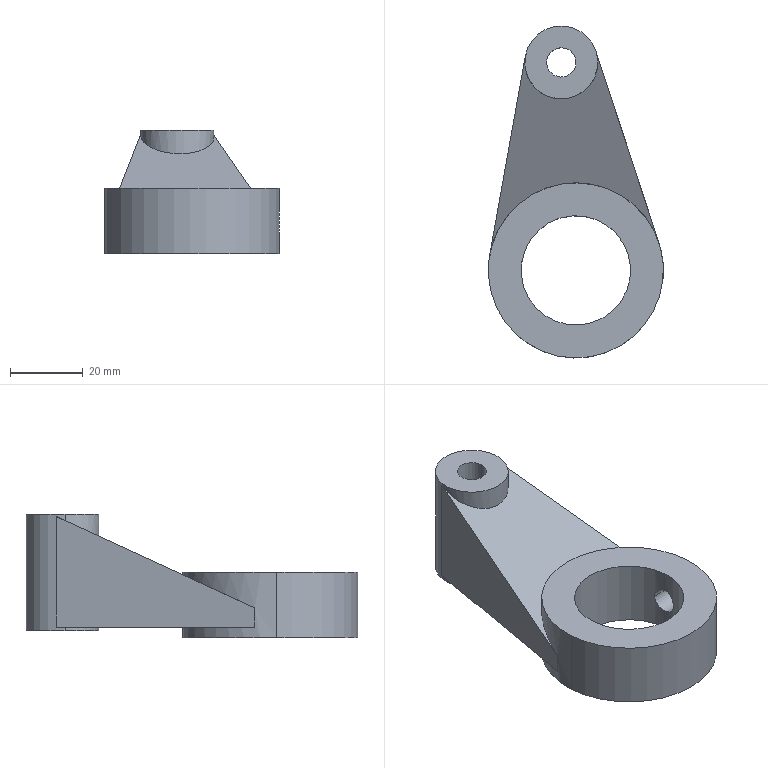Component | SolidWorks | 15Lever-1 | 1 solid | 26 faces | box 48 x 91 x 34 mm | volume 35312 mm3 | cylinder 13 | plane 13 | commonest cylinder face diameters 20 x3 6.8 x2 14.5 x2 30 x2 48 x2 8.02 x2
STEP:
#1=COLOUR_RGB('',0.7922,0.8196,0.9333);
#2=FILL_AREA_STYLE_COLOUR('',#1);
#3=FILL_AREA_STYLE('',(#2));
#4=SURFACE_STYLE_FILL_AREA(#3);
#5=SURFACE_SIDE_STYLE('',(#4));
#6=SURFACE_STYLE_USAGE(.BOTH.,#5);
#7=PRESENTATION_STYLE_ASSIGNMENT((#6));
#8=CARTESIAN_POINT('',(2.078,-2.267,14.724));
#9=VERTEX_POINT('',#8);
#10=CARTESIAN_POINT('',(2.083,-2.133,14.591));
#11=VERTEX_POINT('',#10);
#12=CARTESIAN_POINT('',(2.078,-2.267,14.724));
#13=CARTESIAN_POINT('',(2.078,-2.267,14.716));
#14=CARTESIAN_POINT('',(2.078,-2.267,14.707));
#15=CARTESIAN_POINT('',(2.078,-2.263,14.69));
#16=CARTESIAN_POINT('',(2.079,-2.26,14.681));
#17=CARTESIAN_POINT('',(2.08,-2.254,14.665));
#18=CARTESIAN_POINT('',(2.08,-2.25,14.657));
#19=CARTESIAN_POINT('',(2.081,-2.24,14.643));
#20=CARTESIAN_POINT('',(2.082,-2.234,14.636));
#21=CARTESIAN_POINT('',(2.083,-2.222,14.624));
#22=CARTESIAN_POINT('',(2.084,-2.215,14.618));
#23=CARTESIAN_POINT('',(2.084,-2.2,14.608));
#24=CARTESIAN_POINT('',(2.085,-2.192,14.604));
#25=CARTESIAN_POINT('',(2.085,-2.176,14.597));
#26=CARTESIAN_POINT('',(2.085,-2.168,14.595));
#27=CARTESIAN_POINT('',(2.085,-2.15,14.591));
#28=CARTESIAN_POINT('',(2.084,-2.142,14.591));
#29=CARTESIAN_POINT('',(2.083,-2.133,14.591));
#30=B_SPLINE_CURVE_WITH_KNOTS('',3,(#12,#13,#14,#15,#16,#17,#18,#19,#20,#21,#22,#23,#24,#25,#26,#27,#28,#29),.UNSPECIFIED.,.F.,.F.,(4,2,2,2,2,2,2,2,4),(0.016,0.01666,0.01733,0.018,0.01866,0.01933,0.01999,0.02066,0.02133),.UNSPECIFIED.);
#31=EDGE_CURVE('',#9,#11,#30,.T.);
#32=ORIENTED_EDGE('',*,*,#31,.F.);
#33=CARTESIAN_POINT('',(2.437,-2.242,14.724));
#34=VERTEX_POINT('',#33);
#35=CARTESIAN_POINT('',(2.446,-2.242,14.724));
#36=DIRECTION('',(0.9975,0.07,0.));
#37=VECTOR('',#36,39.37);
#38=LINE('',#35,#37);
#39=EDGE_CURVE('',#9,#34,#38,.T.);
#40=ORIENTED_EDGE('',*,*,#39,.T.);
#41=CARTESIAN_POINT('',(2.437,-2.108,14.591));
#42=VERTEX_POINT('',#41);
#43=CARTESIAN_POINT('',(2.437,-2.242,14.724));
#44=CARTESIAN_POINT('',(2.437,-2.242,14.716));
#45=CARTESIAN_POINT('',(2.437,-2.241,14.707));
#46=CARTESIAN_POINT('',(2.437,-2.238,14.69));
#47=CARTESIAN_POINT('',(2.437,-2.235,14.681));
#48=CARTESIAN_POINT('',(2.438,-2.229,14.665));
#49=CARTESIAN_POINT('',(2.438,-2.224,14.657));
#50=CARTESIAN_POINT('',(2.438,-2.215,14.643));
#51=CARTESIAN_POINT('',(2.439,-2.209,14.636));
#52=CARTESIAN_POINT('',(2.439,-2.197,14.624));
#53=CARTESIAN_POINT('',(2.439,-2.19,14.618));
#54=CARTESIAN_POINT('',(2.439,-2.175,14.608));
#55=CARTESIAN_POINT('',(2.439,-2.167,14.604));
#56=CARTESIAN_POINT('',(2.439,-2.151,14.597));
#57=CARTESIAN_POINT('',(2.439,-2.143,14.595));
#58=CARTESIAN_POINT('',(2.438,-2.126,14.591));
#59=CARTESIAN_POINT('',(2.438,-2.117,14.591));
#60=CARTESIAN_POINT('',(2.437,-2.108,14.591));
#61=B_SPLINE_CURVE_WITH_KNOTS('',3,(#43,#44,#45,#46,#47,#48,#49,#50,#51,#52,#53,#54,#55,#56,#57,#58,#59,#60),.UNSPECIFIED.,.F.,.F.,(4,2,2,2,2,2,2,2,4),(0.01064,0.01131,0.01197,0.01264,0.0133,0.01397,0.01464,0.0153,0.01597),.UNSPECIFIED.);
#62=EDGE_CURVE('',#34,#42,#61,.T.);
#63=ORIENTED_EDGE('',*,*,#62,.T.);
#64=CARTESIAN_POINT('',(2.418,-1.975,14.724));
#65=VERTEX_POINT('',#64);
#66=CARTESIAN_POINT('',(2.437,-2.108,14.591));
#67=CARTESIAN_POINT('',(2.436,-2.099,14.591));
#68=CARTESIAN_POINT('',(2.436,-2.091,14.591));
#69=CARTESIAN_POINT('',(2.434,-2.073,14.595));
#70=CARTESIAN_POINT('',(2.433,-2.065,14.597));
#71=CARTESIAN_POINT('',(2.431,-2.049,14.604));
#72=CARTESIAN_POINT('',(2.43,-2.041,14.608));
#73=CARTESIAN_POINT('',(2.428,-2.027,14.618));
#74=CARTESIAN_POINT('',(2.427,-2.02,14.624));
#75=CARTESIAN_POINT('',(2.425,-2.008,14.636));
#76=CARTESIAN_POINT('',(2.424,-2.002,14.643));
#77=CARTESIAN_POINT('',(2.422,-1.993,14.657));
#78=CARTESIAN_POINT('',(2.421,-1.989,14.665));
#79=CARTESIAN_POINT('',(2.42,-1.982,14.681));
#80=CARTESIAN_POINT('',(2.419,-1.979,14.69));
#81=CARTESIAN_POINT('',(2.418,-1.976,14.707));
#82=CARTESIAN_POINT('',(2.418,-1.975,14.716));
#83=CARTESIAN_POINT('',(2.418,-1.975,14.724));
#84=B_SPLINE_CURVE_WITH_KNOTS('',3,(#66,#67,#68,#69,#70,#71,#72,#73,#74,#75,#76,#77,#78,#79,#80,#81,#82,#83),.UNSPECIFIED.,.F.,.F.,(4,2,2,2,2,2,2,2,4),(0.01597,0.01663,0.0173,0.01796,0.01863,0.01929,0.01995,0.02062,0.02128),.UNSPECIFIED.);
#85=EDGE_CURVE('',#42,#65,#84,.T.);
#86=ORIENTED_EDGE('',*,*,#85,.T.);
#87=CARTESIAN_POINT('',(2.059,-2.,14.724));
#88=VERTEX_POINT('',#87);
#89=CARTESIAN_POINT('',(2.428,-1.974,14.724));
#90=DIRECTION('',(0.9975,0.07,0.));
#91=VECTOR('',#90,39.37);
#92=LINE('',#89,#91);
#93=EDGE_CURVE('',#88,#65,#92,.T.);
#94=ORIENTED_EDGE('',*,*,#93,.F.);
#95=CARTESIAN_POINT('',(2.083,-2.133,14.591));
#96=CARTESIAN_POINT('',(2.083,-2.124,14.591));
#97=CARTESIAN_POINT('',(2.082,-2.115,14.591));
#98=CARTESIAN_POINT('',(2.08,-2.098,14.595));
#99=CARTESIAN_POINT('',(2.079,-2.09,14.597));
#100=CARTESIAN_POINT('',(2.076,-2.074,14.604));
#101=CARTESIAN_POINT('',(2.075,-2.066,14.608));
#102=CARTESIAN_POINT('',(2.072,-2.052,14.618));
#103=CARTESIAN_POINT('',(2.071,-2.045,14.624));
#104=CARTESIAN_POINT('',(2.068,-2.033,14.636));
#105=CARTESIAN_POINT('',(2.066,-2.027,14.643));
#106=CARTESIAN_POINT('',(2.064,-2.018,14.657));
#107=CARTESIAN_POINT('',(2.063,-2.014,14.665));
#108=CARTESIAN_POINT('',(2.061,-2.007,14.681));
#109=CARTESIAN_POINT('',(2.06,-2.005,14.69));
#110=CARTESIAN_POINT('',(2.059,-2.001,14.707));
#111=CARTESIAN_POINT('',(2.059,-2.,14.716));
#112=CARTESIAN_POINT('',(2.059,-2.,14.724));
#113=B_SPLINE_CURVE_WITH_KNOTS('',3,(#95,#96,#97,#98,#99,#100,#101,#102,#103,#104,#105,#106,#107,#108,#109,#110,#111,#112),.UNSPECIFIED.,.F.,.F.,(4,2,2,2,2,2,2,2,4),(0.,0.0006667,0.001333,0.002,0.002667,0.003334,0.004,0.004667,0.005334),.UNSPECIFIED.);
#114=EDGE_CURVE('',#11,#88,#113,.T.);
#115=ORIENTED_EDGE('',*,*,#114,.F.);
#116=EDGE_LOOP('',(#32,#40,#63,#86,#94,#115));
#117=FACE_OUTER_BOUND('',#116,.T.);
#118=CARTESIAN_POINT('',(2.437,-2.108,14.724));
#119=DIRECTION('',(0.9975,0.07,0.));
#120=DIRECTION('',(-0.07,0.9975,0.));
#121=AXIS2_PLACEMENT_3D('',#118,#119,#120);
#122=CYLINDRICAL_SURFACE('',#121,0.1339);
#123=ADVANCED_FACE('',(#117),#122,.F.);
#124=CARTESIAN_POINT('',(1.622,0.0899,15.433));
#125=VERTEX_POINT('',#124);
#126=CARTESIAN_POINT('',(1.052,0.04993,15.433));
#127=VERTEX_POINT('',#126);
#128=CARTESIAN_POINT('',(1.337,0.06992,15.433));
#129=DIRECTION('',(0.,-0.,-1.));
#130=DIRECTION('',(-0.9975,-0.07,0.));
#131=AXIS2_PLACEMENT_3D('',#128,#129,#130);
#132=CIRCLE('',#131,0.2854);
#133=EDGE_CURVE('',#125,#127,#132,.T.);
#134=ORIENTED_EDGE('',*,*,#133,.F.);
#135=CARTESIAN_POINT('',(1.622,0.0899,14.449));
#136=VERTEX_POINT('',#135);
#137=CARTESIAN_POINT('',(1.622,0.0899,15.433));
#138=DIRECTION('',(0.,-0.,-1.));
#139=VECTOR('',#138,39.37);
#140=LINE('',#137,#139);
#141=EDGE_CURVE('',#125,#136,#140,.T.);
#142=ORIENTED_EDGE('',*,*,#141,.T.);
#143=CARTESIAN_POINT('',(1.052,0.04993,14.449));
#144=VERTEX_POINT('',#143);
#145=CARTESIAN_POINT('',(1.337,0.06992,14.449));
#146=DIRECTION('',(0.,-0.,-1.));
#147=DIRECTION('',(-0.9975,-0.07,0.));
#148=AXIS2_PLACEMENT_3D('',#145,#146,#147);
#149=CIRCLE('',#148,0.2854);
#150=EDGE_CURVE('',#136,#144,#149,.T.);
#151=ORIENTED_EDGE('',*,*,#150,.T.);
#152=CARTESIAN_POINT('',(1.052,0.04993,15.433));
#153=DIRECTION('',(0.,-0.,-1.));
#154=VECTOR('',#153,39.37);
#155=LINE('',#152,#154);
#156=EDGE_CURVE('',#127,#144,#155,.T.);
#157=ORIENTED_EDGE('',*,*,#156,.F.);
#158=EDGE_LOOP('',(#134,#142,#151,#157));
#159=FACE_OUTER_BOUND('',#158,.T.);
#160=CARTESIAN_POINT('',(1.337,0.06992,15.433));
#161=DIRECTION('',(0.,-0.,-1.));
#162=DIRECTION('',(-0.9975,-0.07,0.));
#163=AXIS2_PLACEMENT_3D('',#160,#161,#162);
#164=CYLINDRICAL_SURFACE('',#163,0.2854);
#165=ADVANCED_FACE('',(#159),#164,.F.);
#166=CARTESIAN_POINT('',(0.9053,-2.216,14.37));
#167=VERTEX_POINT('',#166);
#168=CARTESIAN_POINT('',(2.083,-2.133,14.37));
#169=VERTEX_POINT('',#168);
#170=CARTESIAN_POINT('',(1.494,-2.174,14.37));
#171=DIRECTION('',(-0.,0.,1.));
#172=DIRECTION('',(0.9975,0.07,0.));
#173=AXIS2_PLACEMENT_3D('',#170,#171,#172);
#174=CIRCLE('',#173,0.5906);
#175=EDGE_CURVE('',#167,#169,#174,.T.);
#176=ORIENTED_EDGE('',*,*,#175,.F.);
#177=CARTESIAN_POINT('',(0.9053,-2.216,15.079));
#178=VERTEX_POINT('',#177);
#179=CARTESIAN_POINT('',(0.9053,-2.216,14.37));
#180=DIRECTION('',(-0.,0.,1.));
#181=VECTOR('',#180,39.37);
#182=LINE('',#179,#181);
#183=EDGE_CURVE('',#167,#178,#182,.T.);
#184=ORIENTED_EDGE('',*,*,#183,.T.);
#185=CARTESIAN_POINT('',(2.083,-2.133,15.079));
#186=VERTEX_POINT('',#185);
#187=CARTESIAN_POINT('',(1.494,-2.174,15.079));
#188=DIRECTION('',(0.,-0.,-1.));
#189=DIRECTION('',(-0.9975,-0.07,0.));
#190=AXIS2_PLACEMENT_3D('',#187,#188,#189);
#191=CIRCLE('',#190,0.5906);
#192=EDGE_CURVE('',#186,#178,#191,.T.);
#193=ORIENTED_EDGE('',*,*,#192,.F.);
#194=CARTESIAN_POINT('',(2.083,-2.133,14.858));
#195=VERTEX_POINT('',#194);
#196=CARTESIAN_POINT('',(2.083,-2.133,14.37));
#197=DIRECTION('',(-0.,0.,1.));
#198=VECTOR('',#197,39.37);
#199=LINE('',#196,#198);
#200=EDGE_CURVE('',#195,#186,#199,.T.);
#201=ORIENTED_EDGE('',*,*,#200,.F.);
#202=CARTESIAN_POINT('',(2.083,-2.133,14.858));
#203=CARTESIAN_POINT('',(2.084,-2.142,14.858));
#204=CARTESIAN_POINT('',(2.085,-2.15,14.857));
#205=CARTESIAN_POINT('',(2.085,-2.168,14.854));
#206=CARTESIAN_POINT('',(2.085,-2.176,14.851));
#207=CARTESIAN_POINT('',(2.085,-2.192,14.845));
#208=CARTESIAN_POINT('',(2.084,-2.2,14.841));
#209=CARTESIAN_POINT('',(2.084,-2.215,14.831));
#210=CARTESIAN_POINT('',(2.083,-2.222,14.825));
#211=CARTESIAN_POINT('',(2.082,-2.234,14.813));
#212=CARTESIAN_POINT('',(2.081,-2.24,14.806));
#213=CARTESIAN_POINT('',(2.08,-2.249,14.792));
#214=CARTESIAN_POINT('',(2.08,-2.254,14.784));
#215=CARTESIAN_POINT('',(2.078,-2.264,14.76));
#216=CARTESIAN_POINT('',(2.078,-2.267,14.742));
#217=CARTESIAN_POINT('',(2.078,-2.267,14.724));
#218=B_SPLINE_CURVE_WITH_KNOTS('',3,(#202,#203,#204,#205,#206,#207,#208,#209,#210,#211,#212,#213,#214,#215,#216,#217),.UNSPECIFIED.,.F.,.F.,(4,2,2,2,2,2,2,4),(0.01066,0.01133,0.012,0.01266,0.01333,0.014,0.01466,0.016),.UNSPECIFIED.);
#219=EDGE_CURVE('',#195,#9,#218,.T.);
#220=ORIENTED_EDGE('',*,*,#219,.T.);
#221=ORIENTED_EDGE('',*,*,#31,.T.);
#222=CARTESIAN_POINT('',(2.083,-2.133,14.37));
#223=DIRECTION('',(-0.,0.,1.));
#224=VECTOR('',#223,39.37);
#225=LINE('',#222,#224);
#226=EDGE_CURVE('',#169,#11,#225,.T.);
#227=ORIENTED_EDGE('',*,*,#226,.F.);
#228=EDGE_LOOP('',(#176,#184,#193,#201,#220,#221,#227));
#229=FACE_OUTER_BOUND('',#228,.T.);
#230=CARTESIAN_POINT('',(1.494,-2.174,14.37));
#231=DIRECTION('',(-0.,0.,1.));
#232=DIRECTION('',(0.9975,0.07,0.));
#233=AXIS2_PLACEMENT_3D('',#230,#231,#232);
#234=CYLINDRICAL_SURFACE('',#233,0.5906);
#235=ADVANCED_FACE('',(#229),#234,.F.);
#236=CARTESIAN_POINT('',(0.5643,-2.007,14.488));
#237=VERTEX_POINT('',#236);
#238=CARTESIAN_POINT('',(0.86,-1.474,14.488));
#239=VERTEX_POINT('',#238);
#240=CARTESIAN_POINT('',(1.494,-2.174,14.488));
#241=DIRECTION('',(0.,-0.,-1.));
#242=DIRECTION('',(-0.9975,-0.07,0.));
#243=AXIS2_PLACEMENT_3D('',#240,#241,#242);
#244=CIRCLE('',#243,0.9449);
#245=EDGE_CURVE('',#237,#239,#244,.T.);
#246=ORIENTED_EDGE('',*,*,#245,.T.);
#247=CARTESIAN_POINT('',(0.86,-1.474,14.717));
#248=VERTEX_POINT('',#247);
#249=CARTESIAN_POINT('',(0.86,-1.474,16.978));
#250=DIRECTION('',(0.,-0.,-1.));
#251=VECTOR('',#250,39.37);
#252=LINE('',#249,#251);
#253=EDGE_CURVE('',#248,#239,#252,.T.);
#254=ORIENTED_EDGE('',*,*,#253,.F.);
#255=CARTESIAN_POINT('',(2.025,-1.392,14.717));
#256=VERTEX_POINT('',#255);
#257=CARTESIAN_POINT('',(2.025,-1.392,14.717));
#258=CARTESIAN_POINT('',(1.649,-1.137,14.847));
#259=CARTESIAN_POINT('',(1.196,-1.169,14.847));
#260=CARTESIAN_POINT('',(0.86,-1.474,14.717));
#261=(BOUNDED_CURVE()B_SPLINE_CURVE(3,(#257,#258,#259,#260),.UNSPECIFIED.,.F.,.F.)B_SPLINE_CURVE_WITH_KNOTS((4,4),(2.476,3.808),.UNSPECIFIED.)CURVE()GEOMETRIC_REPRESENTATION_ITEM()RATIONAL_B_SPLINE_CURVE((1.,0.8575,0.8575,1.))REPRESENTATION_ITEM(''));
#262=EDGE_CURVE('',#256,#248,#261,.T.);
#263=ORIENTED_EDGE('',*,*,#262,.F.);
#264=CARTESIAN_POINT('',(2.025,-1.392,14.488));
#265=VERTEX_POINT('',#264);
#266=CARTESIAN_POINT('',(2.025,-1.392,16.978));
#267=DIRECTION('',(0.,-0.,-1.));
#268=VECTOR('',#267,39.37);
#269=LINE('',#266,#268);
#270=EDGE_CURVE('',#256,#265,#269,.T.);
#271=ORIENTED_EDGE('',*,*,#270,.T.);
#272=CARTESIAN_POINT('',(2.392,-1.879,14.488));
#273=VERTEX_POINT('',#272);
#274=CARTESIAN_POINT('',(1.494,-2.174,14.488));
#275=DIRECTION('',(0.,-0.,-1.));
#276=DIRECTION('',(-0.9975,-0.07,0.));
#277=AXIS2_PLACEMENT_3D('',#274,#275,#276);
#278=CIRCLE('',#277,0.9449);
#279=EDGE_CURVE('',#265,#273,#278,.T.);
#280=ORIENTED_EDGE('',*,*,#279,.T.);
#281=CARTESIAN_POINT('',(2.392,-1.879,14.695));
#282=VERTEX_POINT('',#281);
#283=CARTESIAN_POINT('',(2.392,-1.879,18.131));
#284=DIRECTION('',(0.,-0.,-1.));
#285=VECTOR('',#284,39.37);
#286=LINE('',#283,#285);
#287=EDGE_CURVE('',#282,#273,#286,.T.);
#288=ORIENTED_EDGE('',*,*,#287,.F.);
#289=CARTESIAN_POINT('',(0.5643,-2.007,14.695));
#290=VERTEX_POINT('',#289);
#291=CARTESIAN_POINT('',(0.5643,-2.007,14.695));
#292=CARTESIAN_POINT('',(0.7814,-0.7971,15.251));
#293=CARTESIAN_POINT('',(2.008,-0.711,15.251));
#294=CARTESIAN_POINT('',(2.392,-1.879,14.695));
#295=(BOUNDED_CURVE()B_SPLINE_CURVE(3,(#291,#292,#293,#294),.UNSPECIFIED.,.F.,.F.)B_SPLINE_CURVE_WITH_KNOTS((4,4),(1.818,4.465),.UNSPECIFIED.)CURVE()GEOMETRIC_REPRESENTATION_ITEM()RATIONAL_B_SPLINE_CURVE((1.,0.4967,0.4967,1.))REPRESENTATION_ITEM(''));
#296=EDGE_CURVE('',#290,#282,#295,.T.);
#297=ORIENTED_EDGE('',*,*,#296,.F.);
#298=CARTESIAN_POINT('',(0.5643,-2.007,18.131));
#299=DIRECTION('',(0.,-0.,-1.));
#300=VECTOR('',#299,39.37);
#301=LINE('',#298,#300);
#302=EDGE_CURVE('',#290,#237,#301,.T.);
#303=ORIENTED_EDGE('',*,*,#302,.T.);
#304=EDGE_LOOP('',(#246,#254,#263,#271,#280,#288,#297,#303));
#305=FACE_BOUND('',#304,.T.);
#306=CARTESIAN_POINT('',(0.5518,-2.24,15.079));
#307=VERTEX_POINT('',#306);
#308=CARTESIAN_POINT('',(2.437,-2.108,15.079));
#309=VERTEX_POINT('',#308);
#310=CARTESIAN_POINT('',(1.494,-2.174,15.079));
#311=DIRECTION('',(0.,-0.,-1.));
#312=DIRECTION('',(-0.9975,-0.07,0.));
#313=AXIS2_PLACEMENT_3D('',#310,#311,#312);
#314=CIRCLE('',#313,0.9449);
#315=EDGE_CURVE('',#307,#309,#314,.T.);
#316=ORIENTED_EDGE('',*,*,#315,.T.);
#317=CARTESIAN_POINT('',(2.437,-2.108,14.858));
#318=VERTEX_POINT('',#317);
#319=CARTESIAN_POINT('',(2.437,-2.108,15.079));
#320=DIRECTION('',(0.,-0.,-1.));
#321=VECTOR('',#320,39.37);
#322=LINE('',#319,#321);
#323=EDGE_CURVE('',#309,#318,#322,.T.);
#324=ORIENTED_EDGE('',*,*,#323,.T.);
#325=CARTESIAN_POINT('',(2.418,-1.975,14.724));
#326=CARTESIAN_POINT('',(2.418,-1.975,14.733));
#327=CARTESIAN_POINT('',(2.418,-1.976,14.742));
#328=CARTESIAN_POINT('',(2.419,-1.979,14.759));
#329=CARTESIAN_POINT('',(2.42,-1.982,14.768));
#330=CARTESIAN_POINT('',(2.421,-1.989,14.784));
#331=CARTESIAN_POINT('',(2.422,-1.993,14.792));
#332=CARTESIAN_POINT('',(2.424,-2.002,14.806));
#333=CARTESIAN_POINT('',(2.425,-2.008,14.813));
#334=CARTESIAN_POINT('',(2.427,-2.02,14.825));
#335=CARTESIAN_POINT('',(2.428,-2.027,14.831));
#336=CARTESIAN_POINT('',(2.43,-2.041,14.841));
#337=CARTESIAN_POINT('',(2.431,-2.049,14.845));
#338=CARTESIAN_POINT('',(2.433,-2.065,14.851));
#339=CARTESIAN_POINT('',(2.434,-2.073,14.854));
#340=CARTESIAN_POINT('',(2.436,-2.091,14.857));
#341=CARTESIAN_POINT('',(2.436,-2.099,14.858));
#342=CARTESIAN_POINT('',(2.437,-2.108,14.858));
#343=B_SPLINE_CURVE_WITH_KNOTS('',3,(#325,#326,#327,#328,#329,#330,#331,#332,#333,#334,#335,#336,#337,#338,#339,#340,#341,#342),.UNSPECIFIED.,.F.,.F.,(4,2,2,2,2,2,2,2,4),(0.,0.0006654,0.001331,0.001996,0.002661,0.003327,0.003992,0.004658,0.005323),.UNSPECIFIED.);
#344=EDGE_CURVE('',#65,#318,#343,.T.);
#345=ORIENTED_EDGE('',*,*,#344,.F.);
#346=ORIENTED_EDGE('',*,*,#85,.F.);
#347=CARTESIAN_POINT('',(2.437,-2.108,14.37));
#348=VERTEX_POINT('',#347);
#349=CARTESIAN_POINT('',(2.437,-2.108,15.079));
#350=DIRECTION('',(0.,-0.,-1.));
#351=VECTOR('',#350,39.37);
#352=LINE('',#349,#351);
#353=EDGE_CURVE('',#42,#348,#352,.T.);
#354=ORIENTED_EDGE('',*,*,#353,.T.);
#355=CARTESIAN_POINT('',(0.5518,-2.24,14.37));
#356=VERTEX_POINT('',#355);
#357=CARTESIAN_POINT('',(1.494,-2.174,14.37));
#358=DIRECTION('',(0.,-0.,-1.));
#359=DIRECTION('',(-0.9975,-0.07,0.));
#360=AXIS2_PLACEMENT_3D('',#357,#358,#359);
#361=CIRCLE('',#360,0.9449);
#362=EDGE_CURVE('',#356,#348,#361,.T.);
#363=ORIENTED_EDGE('',*,*,#362,.F.);
#364=CARTESIAN_POINT('',(0.5518,-2.24,15.079));
#365=DIRECTION('',(0.,-0.,-1.));
#366=VECTOR('',#365,39.37);
#367=LINE('',#364,#366);
#368=EDGE_CURVE('',#307,#356,#367,.T.);
#369=ORIENTED_EDGE('',*,*,#368,.F.);
#370=EDGE_LOOP('',(#316,#324,#345,#346,#354,#363,#369));
#371=FACE_OUTER_BOUND('',#370,.T.);
#372=CARTESIAN_POINT('',(1.494,-2.174,15.079));
#373=DIRECTION('',(0.,-0.,-1.));
#374=DIRECTION('',(-0.9975,-0.07,0.));
#375=AXIS2_PLACEMENT_3D('',#372,#373,#374);
#376=CYLINDRICAL_SURFACE('',#375,0.9449);
#377=ADVANCED_FACE('',(#305,#371),#376,.T.);
#378=CARTESIAN_POINT('',(1.73,0.09748,15.709));
#379=VERTEX_POINT('',#378);
#380=CARTESIAN_POINT('',(0.9442,0.04236,15.709));
#381=VERTEX_POINT('',#380);
#382=CARTESIAN_POINT('',(1.337,0.06992,15.709));
#383=DIRECTION('',(-0.,0.,1.));
#384=DIRECTION('',(0.9975,0.07,0.));
#385=AXIS2_PLACEMENT_3D('',#382,#383,#384);
#386=CIRCLE('',#385,0.3937);
#387=EDGE_CURVE('',#379,#381,#386,.T.);
#388=ORIENTED_EDGE('',*,*,#387,.F.);
#389=CARTESIAN_POINT('',(1.73,0.09748,15.636));
#390=VERTEX_POINT('',#389);
#391=CARTESIAN_POINT('',(1.73,0.09748,15.709));
#392=DIRECTION('',(0.,-0.,-1.));
#393=VECTOR('',#392,39.37);
#394=LINE('',#391,#393);
#395=EDGE_CURVE('',#379,#390,#394,.T.);
#396=ORIENTED_EDGE('',*,*,#395,.T.);
#397=CARTESIAN_POINT('',(1.711,0.1929,15.681));
#398=VERTEX_POINT('',#397);
#399=CARTESIAN_POINT('',(1.711,0.1929,15.681));
#400=CARTESIAN_POINT('',(1.721,0.1619,15.667));
#401=CARTESIAN_POINT('',(1.727,0.13,15.652));
#402=CARTESIAN_POINT('',(1.73,0.09748,15.636));
#403=(BOUNDED_CURVE()B_SPLINE_CURVE(3,(#399,#400,#401,#402),.UNSPECIFIED.,.F.,.F.)B_SPLINE_CURVE_WITH_KNOTS((4,4),(4.465,4.712),.UNSPECIFIED.)CURVE()GEOMETRIC_REPRESENTATION_ITEM()RATIONAL_B_SPLINE_CURVE((1.,0.9949,0.9949,1.))REPRESENTATION_ITEM(''));
#404=EDGE_CURVE('',#398,#390,#403,.T.);
#405=ORIENTED_EDGE('',*,*,#404,.F.);
#406=CARTESIAN_POINT('',(1.711,0.1929,14.488));
#407=VERTEX_POINT('',#406);
#408=CARTESIAN_POINT('',(1.711,0.1929,18.131));
#409=DIRECTION('',(0.,-0.,-1.));
#410=VECTOR('',#409,39.37);
#411=LINE('',#408,#410);
#412=EDGE_CURVE('',#398,#407,#411,.T.);
#413=ORIENTED_EDGE('',*,*,#412,.T.);
#414=CARTESIAN_POINT('',(1.73,0.09748,14.488));
#415=VERTEX_POINT('',#414);
#416=CARTESIAN_POINT('',(1.337,0.06992,14.488));
#417=DIRECTION('',(0.,-0.,-1.));
#418=DIRECTION('',(-0.9975,-0.07,0.));
#419=AXIS2_PLACEMENT_3D('',#416,#417,#418);
#420=CIRCLE('',#419,0.3937);
#421=EDGE_CURVE('',#407,#415,#420,.T.);
#422=ORIENTED_EDGE('',*,*,#421,.T.);
#423=CARTESIAN_POINT('',(1.73,0.09748,14.449));
#424=VERTEX_POINT('',#423);
#425=CARTESIAN_POINT('',(1.73,0.09748,15.709));
#426=DIRECTION('',(0.,-0.,-1.));
#427=VECTOR('',#426,39.37);
#428=LINE('',#425,#427);
#429=EDGE_CURVE('',#415,#424,#428,.T.);
#430=ORIENTED_EDGE('',*,*,#429,.T.);
#431=CARTESIAN_POINT('',(0.9442,0.04236,14.449));
#432=VERTEX_POINT('',#431);
#433=CARTESIAN_POINT('',(1.337,0.06992,14.449));
#434=DIRECTION('',(-0.,0.,1.));
#435=DIRECTION('',(0.9975,0.07,0.));
#436=AXIS2_PLACEMENT_3D('',#433,#434,#435);
#437=CIRCLE('',#436,0.3937);
#438=EDGE_CURVE('',#424,#432,#437,.T.);
#439=ORIENTED_EDGE('',*,*,#438,.T.);
#440=CARTESIAN_POINT('',(0.9442,0.04236,14.488));
#441=VERTEX_POINT('',#440);
#442=CARTESIAN_POINT('',(0.9442,0.04236,15.709));
#443=DIRECTION('',(0.,-0.,-1.));
#444=VECTOR('',#443,39.37);
#445=LINE('',#442,#444);
#446=EDGE_CURVE('',#441,#432,#445,.T.);
#447=ORIENTED_EDGE('',*,*,#446,.F.);
#448=CARTESIAN_POINT('',(0.9494,0.1394,14.488));
#449=VERTEX_POINT('',#448);
#450=CARTESIAN_POINT('',(1.337,0.06992,14.488));
#451=DIRECTION('',(0.,-0.,-1.));
#452=DIRECTION('',(-0.9975,-0.07,0.));
#453=AXIS2_PLACEMENT_3D('',#450,#451,#452);
#454=CIRCLE('',#453,0.3937);
#455=EDGE_CURVE('',#441,#449,#454,.T.);
#456=ORIENTED_EDGE('',*,*,#455,.T.);
#457=CARTESIAN_POINT('',(0.9494,0.1394,15.681));
#458=VERTEX_POINT('',#457);
#459=CARTESIAN_POINT('',(0.9494,0.1394,18.131));
#460=DIRECTION('',(0.,-0.,-1.));
#461=VECTOR('',#460,39.37);
#462=LINE('',#459,#461);
#463=EDGE_CURVE('',#458,#449,#462,.T.);
#464=ORIENTED_EDGE('',*,*,#463,.F.);
#465=CARTESIAN_POINT('',(0.9442,0.04236,15.636));
#466=VERTEX_POINT('',#465);
#467=CARTESIAN_POINT('',(0.9442,0.04236,15.636));
#468=CARTESIAN_POINT('',(0.9419,0.07484,15.652));
#469=CARTESIAN_POINT('',(0.9436,0.1074,15.667));
#470=CARTESIAN_POINT('',(0.9494,0.1394,15.681));
#471=(BOUNDED_CURVE()B_SPLINE_CURVE(3,(#467,#468,#469,#470),.UNSPECIFIED.,.F.,.F.)B_SPLINE_CURVE_WITH_KNOTS((4,4),(1.571,1.818),.UNSPECIFIED.)CURVE()GEOMETRIC_REPRESENTATION_ITEM()RATIONAL_B_SPLINE_CURVE((1.,0.9949,0.9949,1.))REPRESENTATION_ITEM(''));
#472=EDGE_CURVE('',#466,#458,#471,.T.);
#473=ORIENTED_EDGE('',*,*,#472,.F.);
#474=CARTESIAN_POINT('',(0.9442,0.04236,15.709));
#475=DIRECTION('',(0.,-0.,-1.));
#476=VECTOR('',#475,39.37);
#477=LINE('',#474,#476);
#478=EDGE_CURVE('',#381,#466,#477,.T.);
#479=ORIENTED_EDGE('',*,*,#478,.F.);
#480=EDGE_LOOP('',(#388,#396,#405,#413,#422,#430,#439,#447,#456,#464,#473,#479));
#481=FACE_OUTER_BOUND('',#480,.T.);
#482=CARTESIAN_POINT('',(1.337,0.06992,15.709));
#483=DIRECTION('',(0.,-0.,-1.));
#484=DIRECTION('',(-0.9975,-0.07,0.));
#485=AXIS2_PLACEMENT_3D('',#482,#483,#484);
#486=CYLINDRICAL_SURFACE('',#485,0.3937);
#487=ADVANCED_FACE('',(#481),#486,.T.);
#488=ORIENTED_EDGE('',*,*,#395,.F.);
#489=CARTESIAN_POINT('',(1.337,0.06992,15.709));
#490=DIRECTION('',(-0.,0.,1.));
#491=DIRECTION('',(0.9975,0.07,0.));
#492=AXIS2_PLACEMENT_3D('',#489,#490,#491);
#493=CIRCLE('',#492,0.3937);
#494=EDGE_CURVE('',#381,#379,#493,.T.);
#495=ORIENTED_EDGE('',*,*,#494,.F.);
#496=ORIENTED_EDGE('',*,*,#478,.T.);
#497=CARTESIAN_POINT('',(1.73,0.09748,15.636));
#498=CARTESIAN_POINT('',(1.785,-0.688,15.269));
#499=CARTESIAN_POINT('',(0.9993,-0.7431,15.269));
#500=CARTESIAN_POINT('',(0.9442,0.04236,15.636));
#501=(BOUNDED_CURVE()B_SPLINE_CURVE(3,(#497,#498,#499,#500),.UNSPECIFIED.,.F.,.F.)B_SPLINE_CURVE_WITH_KNOTS((4,4),(4.712,7.854),.UNSPECIFIED.)CURVE()GEOMETRIC_REPRESENTATION_ITEM()RATIONAL_B_SPLINE_CURVE((1.,0.3333,0.3333,1.))REPRESENTATION_ITEM(''));
#502=EDGE_CURVE('',#390,#466,#501,.T.);
#503=ORIENTED_EDGE('',*,*,#502,.F.);
#504=EDGE_LOOP('',(#488,#495,#496,#503));
#505=FACE_OUTER_BOUND('',#504,.T.);
#506=CARTESIAN_POINT('',(1.337,0.06992,15.709));
#507=DIRECTION('',(0.,-0.,-1.));
#508=DIRECTION('',(-0.9975,-0.07,0.));
#509=AXIS2_PLACEMENT_3D('',#506,#507,#508);
#510=CYLINDRICAL_SURFACE('',#509,0.3937);
#511=ADVANCED_FACE('',(#505),#510,.T.);
#512=CARTESIAN_POINT('',(1.179,0.05886,15.433));
#513=VERTEX_POINT('',#512);
#514=CARTESIAN_POINT('',(1.494,0.08097,15.433));
#515=VERTEX_POINT('',#514);
#516=CARTESIAN_POINT('',(1.337,0.06992,15.433));
#517=DIRECTION('',(-0.,0.,1.));
#518=DIRECTION('',(-0.9975,-0.07,0.));
#519=AXIS2_PLACEMENT_3D('',#516,#517,#518);
#520=CIRCLE('',#519,0.1579);
#521=EDGE_CURVE('',#513,#515,#520,.T.);
#522=ORIENTED_EDGE('',*,*,#521,.F.);
#523=CARTESIAN_POINT('',(1.179,0.05886,15.709));
#524=VERTEX_POINT('',#523);
#525=CARTESIAN_POINT('',(1.179,0.05886,14.37));
#526=DIRECTION('',(-0.,0.,1.));
#527=VECTOR('',#526,39.37);
#528=LINE('',#525,#527);
#529=EDGE_CURVE('',#513,#524,#528,.T.);
#530=ORIENTED_EDGE('',*,*,#529,.T.);
#531=CARTESIAN_POINT('',(1.494,0.08097,15.709));
#532=VERTEX_POINT('',#531);
#533=CARTESIAN_POINT('',(1.337,0.06992,15.709));
#534=DIRECTION('',(-0.,0.,1.));
#535=DIRECTION('',(0.9975,0.07,0.));
#536=AXIS2_PLACEMENT_3D('',#533,#534,#535);
#537=CIRCLE('',#536,0.1579);
#538=EDGE_CURVE('',#524,#532,#537,.T.);
#539=ORIENTED_EDGE('',*,*,#538,.T.);
#540=CARTESIAN_POINT('',(1.494,0.08097,14.37));
#541=DIRECTION('',(-0.,0.,1.));
#542=VECTOR('',#541,39.37);
#543=LINE('',#540,#542);
#544=EDGE_CURVE('',#515,#532,#543,.T.);
#545=ORIENTED_EDGE('',*,*,#544,.F.);
#546=EDGE_LOOP('',(#522,#530,#539,#545));
#547=FACE_OUTER_BOUND('',#546,.T.);
#548=CARTESIAN_POINT('',(1.337,0.06992,14.37));
#549=DIRECTION('',(-0.,0.,1.));
#550=DIRECTION('',(0.9975,0.07,0.));
#551=AXIS2_PLACEMENT_3D('',#548,#549,#550);
#552=CYLINDRICAL_SURFACE('',#551,0.1579);
#553=ADVANCED_FACE('',(#547),#552,.F.);
#554=ORIENTED_EDGE('',*,*,#529,.F.);
#555=CARTESIAN_POINT('',(1.337,0.06992,15.433));
#556=DIRECTION('',(-0.,0.,1.));
#557=DIRECTION('',(-0.9975,-0.07,0.));
#558=AXIS2_PLACEMENT_3D('',#555,#556,#557);
#559=CIRCLE('',#558,0.1579);
#560=EDGE_CURVE('',#515,#513,#559,.T.);
#561=ORIENTED_EDGE('',*,*,#560,.F.);
#562=ORIENTED_EDGE('',*,*,#544,.T.);
#563=CARTESIAN_POINT('',(1.337,0.06992,15.709));
#564=DIRECTION('',(-0.,0.,1.));
#565=DIRECTION('',(0.9975,0.07,0.));
#566=AXIS2_PLACEMENT_3D('',#563,#564,#565);
#567=CIRCLE('',#566,0.1579);
#568=EDGE_CURVE('',#532,#524,#567,.T.);
#569=ORIENTED_EDGE('',*,*,#568,.T.);
#570=EDGE_LOOP('',(#554,#561,#562,#569));
#571=FACE_OUTER_BOUND('',#570,.T.);
#572=CARTESIAN_POINT('',(1.337,0.06992,14.37));
#573=DIRECTION('',(-0.,0.,1.));
#574=DIRECTION('',(0.9975,0.07,0.));
#575=AXIS2_PLACEMENT_3D('',#572,#573,#574);
#576=CYLINDRICAL_SURFACE('',#575,0.1579);
#577=ADVANCED_FACE('',(#571),#576,.F.);
#578=ORIENTED_EDGE('',*,*,#279,.F.);
#579=CARTESIAN_POINT('',(1.63,-0.1925,14.488));
#580=VERTEX_POINT('',#579);
#581=CARTESIAN_POINT('',(2.205,-1.941,14.488));
#582=DIRECTION('',(-0.3123,0.95,-0.));
#583=VECTOR('',#582,39.37);
#584=LINE('',#581,#583);
#585=EDGE_CURVE('',#265,#580,#584,.T.);
#586=ORIENTED_EDGE('',*,*,#585,.T.);
#587=CARTESIAN_POINT('',(1.337,0.06992,14.488));
#588=DIRECTION('',(0.,-0.,-1.));
#589=DIRECTION('',(-0.9975,-0.07,0.));
#590=AXIS2_PLACEMENT_3D('',#587,#588,#589);
#591=CIRCLE('',#590,0.3937);
#592=EDGE_CURVE('',#415,#580,#591,.T.);
#593=ORIENTED_EDGE('',*,*,#592,.F.);
#594=ORIENTED_EDGE('',*,*,#421,.F.);
#595=CARTESIAN_POINT('',(2.392,-1.879,14.488));
#596=DIRECTION('',(-0.3123,0.95,-0.));
#597=VECTOR('',#596,39.37);
#598=LINE('',#595,#597);
#599=EDGE_CURVE('',#273,#407,#598,.T.);
#600=ORIENTED_EDGE('',*,*,#599,.F.);
#601=EDGE_LOOP('',(#578,#586,#593,#594,#600));
#602=FACE_OUTER_BOUND('',#601,.T.);
#603=CARTESIAN_POINT('',(1.494,-2.174,14.488));
#604=DIRECTION('',(0.,-0.,-1.));
#605=DIRECTION('',(-0.9975,-0.07,-0.));
#606=AXIS2_PLACEMENT_3D('',#603,#604,#605);
#607=PLANE('',#606);
#608=ADVANCED_FACE('',(#602),#607,.T.);
#609=ORIENTED_EDGE('',*,*,#429,.F.);
#610=ORIENTED_EDGE('',*,*,#592,.T.);
#611=CARTESIAN_POINT('',(1.63,-0.1925,15.287));
#612=VERTEX_POINT('',#611);
#613=CARTESIAN_POINT('',(1.63,-0.1925,16.978));
#614=DIRECTION('',(0.,-0.,-1.));
#615=VECTOR('',#614,39.37);
#616=LINE('',#613,#615);
#617=EDGE_CURVE('',#612,#580,#616,.T.);
#618=ORIENTED_EDGE('',*,*,#617,.F.);
#619=CARTESIAN_POINT('',(1.083,-0.2309,15.287));
#620=VERTEX_POINT('',#619);
#621=CARTESIAN_POINT('',(1.083,-0.2309,15.287));
#622=CARTESIAN_POINT('',(1.255,-0.3763,15.214));
#623=CARTESIAN_POINT('',(1.48,-0.3606,15.214));
#624=CARTESIAN_POINT('',(1.63,-0.1925,15.287));
#625=(BOUNDED_CURVE()B_SPLINE_CURVE(3,(#621,#622,#623,#624),.UNSPECIFIED.,.F.,.T.)B_SPLINE_CURVE_WITH_KNOTS((4,4),(5.512,7.054),.UNSPECIFIED.)CURVE()GEOMETRIC_REPRESENTATION_ITEM()RATIONAL_B_SPLINE_CURVE((1.,0.8114,0.8114,1.))REPRESENTATION_ITEM(''));
#626=EDGE_CURVE('',#620,#612,#625,.T.);
#627=ORIENTED_EDGE('',*,*,#626,.F.);
#628=CARTESIAN_POINT('',(1.083,-0.2309,14.488));
#629=VERTEX_POINT('',#628);
#630=CARTESIAN_POINT('',(1.083,-0.2309,16.978));
#631=DIRECTION('',(0.,-0.,-1.));
#632=VECTOR('',#631,39.37);
#633=LINE('',#630,#632);
#634=EDGE_CURVE('',#620,#629,#633,.T.);
#635=ORIENTED_EDGE('',*,*,#634,.T.);
#636=CARTESIAN_POINT('',(1.337,0.06992,14.488));
#637=DIRECTION('',(0.,-0.,-1.));
#638=DIRECTION('',(-0.9975,-0.07,0.));
#639=AXIS2_PLACEMENT_3D('',#636,#637,#638);
#640=CIRCLE('',#639,0.3937);
#641=EDGE_CURVE('',#629,#441,#640,.T.);
#642=ORIENTED_EDGE('',*,*,#641,.T.);
#643=ORIENTED_EDGE('',*,*,#446,.T.);
#644=CARTESIAN_POINT('',(1.337,0.06992,14.449));
#645=DIRECTION('',(-0.,0.,1.));
#646=DIRECTION('',(0.9975,0.07,0.));
#647=AXIS2_PLACEMENT_3D('',#644,#645,#646);
#648=CIRCLE('',#647,0.3937);
#649=EDGE_CURVE('',#432,#424,#648,.T.);
#650=ORIENTED_EDGE('',*,*,#649,.T.);
#651=EDGE_LOOP('',(#609,#610,#618,#627,#635,#642,#643,#650));
#652=FACE_OUTER_BOUND('',#651,.T.);
#653=CARTESIAN_POINT('',(1.337,0.06992,15.709));
#654=DIRECTION('',(0.,-0.,-1.));
#655=DIRECTION('',(-0.9975,-0.07,0.));
#656=AXIS2_PLACEMENT_3D('',#653,#654,#655);
#657=CYLINDRICAL_SURFACE('',#656,0.3937);
#658=ADVANCED_FACE('',(#652),#657,.T.);
#659=ORIENTED_EDGE('',*,*,#568,.F.);
#660=ORIENTED_EDGE('',*,*,#538,.F.);
#661=EDGE_LOOP('',(#659,#660));
#662=FACE_BOUND('',#661,.T.);
#663=ORIENTED_EDGE('',*,*,#494,.T.);
#664=ORIENTED_EDGE('',*,*,#387,.T.);
#665=EDGE_LOOP('',(#663,#664));
#666=FACE_OUTER_BOUND('',#665,.T.);
#667=CARTESIAN_POINT('',(1.337,0.06992,15.709));
#668=DIRECTION('',(-0.,0.,1.));
#669=DIRECTION('',(0.9975,0.07,0.));
#670=AXIS2_PLACEMENT_3D('',#667,#668,#669);
#671=PLANE('',#670);
#672=ADVANCED_FACE('',(#662,#666),#671,.T.);
#673=CARTESIAN_POINT('',(1.337,0.06992,14.449));
#674=DIRECTION('',(0.,-0.,-1.));
#675=DIRECTION('',(-0.9975,-0.07,0.));
#676=AXIS2_PLACEMENT_3D('',#673,#674,#675);
#677=CIRCLE('',#676,0.2854);
#678=EDGE_CURVE('',#144,#136,#677,.T.);
#679=ORIENTED_EDGE('',*,*,#678,.F.);
#680=ORIENTED_EDGE('',*,*,#150,.F.);
#681=EDGE_LOOP('',(#679,#680));
#682=FACE_BOUND('',#681,.T.);
#683=ORIENTED_EDGE('',*,*,#649,.F.);
#684=ORIENTED_EDGE('',*,*,#438,.F.);
#685=EDGE_LOOP('',(#683,#684));
#686=FACE_OUTER_BOUND('',#685,.T.);
#687=CARTESIAN_POINT('',(1.337,0.06992,14.449));
#688=DIRECTION('',(-0.,0.,1.));
#689=DIRECTION('',(0.9975,0.07,0.));
#690=AXIS2_PLACEMENT_3D('',#687,#688,#689);
#691=PLANE('',#690);
#692=ADVANCED_FACE('',(#682,#686),#691,.F.);
#693=CARTESIAN_POINT('',(0.792,-0.738,15.278));
#694=DIRECTION('',(0.1609,0.8969,0.412));
#695=VECTOR('',#694,39.37);
#696=LINE('',#693,#695);
#697=EDGE_CURVE('',#290,#458,#696,.T.);
#698=ORIENTED_EDGE('',*,*,#697,.F.);
#699=ORIENTED_EDGE('',*,*,#296,.T.);
#700=CARTESIAN_POINT('',(1.989,-0.654,15.278));
#701=DIRECTION('',(-0.2846,0.8656,0.412));
#702=VECTOR('',#701,39.37);
#703=LINE('',#700,#702);
#704=EDGE_CURVE('',#282,#398,#703,.T.);
#705=ORIENTED_EDGE('',*,*,#704,.T.);
#706=ORIENTED_EDGE('',*,*,#404,.T.);
#707=ORIENTED_EDGE('',*,*,#502,.T.);
#708=ORIENTED_EDGE('',*,*,#472,.T.);
#709=EDGE_LOOP('',(#698,#699,#705,#706,#707,#708));
#710=FACE_OUTER_BOUND('',#709,.T.);
#711=CARTESIAN_POINT('',(1.369,-0.3838,15.424));
#712=DIRECTION('',(0.02958,-0.4216,0.9063));
#713=DIRECTION('',(0.06344,-0.9041,-0.4226));
#714=AXIS2_PLACEMENT_3D('',#711,#712,#713);
#715=PLANE('',#714);
#716=ADVANCED_FACE('',(#710),#715,.T.);
#717=CARTESIAN_POINT('',(0.7581,-2.042,14.488));
#718=DIRECTION('',(0.1765,0.9843,0.));
#719=VECTOR('',#718,39.37);
#720=LINE('',#717,#719);
#721=EDGE_CURVE('',#239,#629,#720,.T.);
#722=ORIENTED_EDGE('',*,*,#721,.F.);
#723=ORIENTED_EDGE('',*,*,#245,.F.);
#724=CARTESIAN_POINT('',(0.5643,-2.007,14.488));
#725=DIRECTION('',(0.1765,0.9843,0.));
#726=VECTOR('',#725,39.37);
#727=LINE('',#724,#726);
#728=EDGE_CURVE('',#237,#449,#727,.T.);
#729=ORIENTED_EDGE('',*,*,#728,.T.);
#730=ORIENTED_EDGE('',*,*,#455,.F.);
#731=ORIENTED_EDGE('',*,*,#641,.F.);
#732=EDGE_LOOP('',(#722,#723,#729,#730,#731));
#733=FACE_OUTER_BOUND('',#732,.T.);
#734=CARTESIAN_POINT('',(1.494,-2.174,14.488));
#735=DIRECTION('',(0.,-0.,-1.));
#736=DIRECTION('',(-0.9975,-0.07,-0.));
#737=AXIS2_PLACEMENT_3D('',#734,#735,#736);
#738=PLANE('',#737);
#739=ADVANCED_FACE('',(#733),#738,.T.);
#740=ORIENTED_EDGE('',*,*,#302,.F.);
#741=ORIENTED_EDGE('',*,*,#697,.T.);
#742=ORIENTED_EDGE('',*,*,#463,.T.);
#743=ORIENTED_EDGE('',*,*,#728,.F.);
#744=EDGE_LOOP('',(#740,#741,#742,#743));
#745=FACE_OUTER_BOUND('',#744,.T.);
#746=CARTESIAN_POINT('',(0.5643,-2.007,18.131));
#747=DIRECTION('',(-0.9843,0.1765,-0.));
#748=DIRECTION('',(-0.1765,-0.9843,-0.));
#749=AXIS2_PLACEMENT_3D('',#746,#747,#748);
#750=PLANE('',#749);
#751=ADVANCED_FACE('',(#745),#750,.T.);
#752=ORIENTED_EDGE('',*,*,#704,.F.);
#753=ORIENTED_EDGE('',*,*,#287,.T.);
#754=ORIENTED_EDGE('',*,*,#599,.T.);
#755=ORIENTED_EDGE('',*,*,#412,.F.);
#756=EDGE_LOOP('',(#752,#753,#754,#755));
#757=FACE_OUTER_BOUND('',#756,.T.);
#758=CARTESIAN_POINT('',(2.392,-1.879,18.131));
#759=DIRECTION('',(-0.95,-0.3123,-0.));
#760=DIRECTION('',(0.3123,-0.95,0.));
#761=AXIS2_PLACEMENT_3D('',#758,#759,#760);
#762=PLANE('',#761);
#763=ADVANCED_FACE('',(#757),#762,.F.);
#764=ORIENTED_EDGE('',*,*,#323,.F.);
#765=CARTESIAN_POINT('',(1.494,-2.174,15.079));
#766=DIRECTION('',(0.,-0.,-1.));
#767=DIRECTION('',(-0.9975,-0.07,0.));
#768=AXIS2_PLACEMENT_3D('',#765,#766,#767);
#769=CIRCLE('',#768,0.9449);
#770=EDGE_CURVE('',#309,#307,#769,.T.);
#771=ORIENTED_EDGE('',*,*,#770,.T.);
#772=ORIENTED_EDGE('',*,*,#368,.T.);
#773=CARTESIAN_POINT('',(1.494,-2.174,14.37));
#774=DIRECTION('',(0.,-0.,-1.));
#775=DIRECTION('',(-0.9975,-0.07,0.));
#776=AXIS2_PLACEMENT_3D('',#773,#774,#775);
#777=CIRCLE('',#776,0.9449);
#778=EDGE_CURVE('',#348,#356,#777,.T.);
#779=ORIENTED_EDGE('',*,*,#778,.F.);
#780=ORIENTED_EDGE('',*,*,#353,.F.);
#781=ORIENTED_EDGE('',*,*,#62,.F.);
#782=CARTESIAN_POINT('',(2.437,-2.108,14.858));
#783=CARTESIAN_POINT('',(2.438,-2.117,14.858));
#784=CARTESIAN_POINT('',(2.438,-2.126,14.857));
#785=CARTESIAN_POINT('',(2.439,-2.143,14.854));
#786=CARTESIAN_POINT('',(2.439,-2.151,14.851));
#787=CARTESIAN_POINT('',(2.439,-2.167,14.845));
#788=CARTESIAN_POINT('',(2.439,-2.175,14.841));
#789=CARTESIAN_POINT('',(2.439,-2.19,14.831));
#790=CARTESIAN_POINT('',(2.439,-2.197,14.825));
#791=CARTESIAN_POINT('',(2.439,-2.209,14.813));
#792=CARTESIAN_POINT('',(2.438,-2.215,14.806));
#793=CARTESIAN_POINT('',(2.438,-2.224,14.792));
#794=CARTESIAN_POINT('',(2.438,-2.229,14.784));
#795=CARTESIAN_POINT('',(2.437,-2.235,14.768));
#796=CARTESIAN_POINT('',(2.437,-2.238,14.759));
#797=CARTESIAN_POINT('',(2.437,-2.241,14.742));
#798=CARTESIAN_POINT('',(2.437,-2.242,14.733));
#799=CARTESIAN_POINT('',(2.437,-2.242,14.724));
#800=B_SPLINE_CURVE_WITH_KNOTS('',3,(#782,#783,#784,#785,#786,#787,#788,#789,#790,#791,#792,#793,#794,#795,#796,#797,#798,#799),.UNSPECIFIED.,.F.,.F.,(4,2,2,2,2,2,2,2,4),(0.005323,0.005988,0.006653,0.007318,0.007983,0.008648,0.009313,0.009978,0.01064),.UNSPECIFIED.);
#801=EDGE_CURVE('',#318,#34,#800,.T.);
#802=ORIENTED_EDGE('',*,*,#801,.F.);
#803=EDGE_LOOP('',(#764,#771,#772,#779,#780,#781,#802));
#804=FACE_OUTER_BOUND('',#803,.T.);
#805=CARTESIAN_POINT('',(1.494,-2.174,15.079));
#806=DIRECTION('',(0.,-0.,-1.));
#807=DIRECTION('',(-0.9975,-0.07,0.));
#808=AXIS2_PLACEMENT_3D('',#805,#806,#807);
#809=CYLINDRICAL_SURFACE('',#808,0.9449);
#810=ADVANCED_FACE('',(#804),#809,.T.);
#811=ORIENTED_EDGE('',*,*,#192,.T.);
#812=CARTESIAN_POINT('',(1.494,-2.174,15.079));
#813=DIRECTION('',(0.,-0.,-1.));
#814=DIRECTION('',(-0.9975,-0.07,0.));
#815=AXIS2_PLACEMENT_3D('',#812,#813,#814);
#816=CIRCLE('',#815,0.5906);
#817=EDGE_CURVE('',#178,#186,#816,.T.);
#818=ORIENTED_EDGE('',*,*,#817,.T.);
#819=EDGE_LOOP('',(#811,#818));
#820=FACE_BOUND('',#819,.T.);
#821=ORIENTED_EDGE('',*,*,#315,.F.);
#822=ORIENTED_EDGE('',*,*,#770,.F.);
#823=EDGE_LOOP('',(#821,#822));
#824=FACE_OUTER_BOUND('',#823,.T.);
#825=CARTESIAN_POINT('',(1.494,-2.174,15.079));
#826=DIRECTION('',(0.,-0.,-1.));
#827=DIRECTION('',(-0.9975,-0.07,-0.));
#828=AXIS2_PLACEMENT_3D('',#825,#826,#827);
#829=PLANE('',#828);
#830=ADVANCED_FACE('',(#820,#824),#829,.F.);
#831=CARTESIAN_POINT('',(1.494,-2.174,14.37));
#832=DIRECTION('',(-0.,0.,1.));
#833=DIRECTION('',(0.9975,0.07,0.));
#834=AXIS2_PLACEMENT_3D('',#831,#832,#833);
#835=CIRCLE('',#834,0.5906);
#836=EDGE_CURVE('',#169,#167,#835,.T.);
#837=ORIENTED_EDGE('',*,*,#836,.T.);
#838=ORIENTED_EDGE('',*,*,#175,.T.);
#839=EDGE_LOOP('',(#837,#838));
#840=FACE_BOUND('',#839,.T.);
#841=ORIENTED_EDGE('',*,*,#362,.T.);
#842=ORIENTED_EDGE('',*,*,#778,.T.);
#843=EDGE_LOOP('',(#841,#842));
#844=FACE_OUTER_BOUND('',#843,.T.);
#845=CARTESIAN_POINT('',(1.494,-2.174,14.37));
#846=DIRECTION('',(0.,-0.,-1.));
#847=DIRECTION('',(-0.9975,-0.07,-0.));
#848=AXIS2_PLACEMENT_3D('',#845,#846,#847);
#849=PLANE('',#848);
#850=ADVANCED_FACE('',(#840,#844),#849,.T.);
#851=ORIENTED_EDGE('',*,*,#262,.T.);
#852=CARTESIAN_POINT('',(1.245,0.6724,15.702));
#853=DIRECTION('',(0.1609,0.8969,0.412));
#854=VECTOR('',#853,39.37);
#855=LINE('',#852,#854);
#856=EDGE_CURVE('',#248,#620,#855,.T.);
#857=ORIENTED_EDGE('',*,*,#856,.T.);
#858=ORIENTED_EDGE('',*,*,#626,.T.);
#859=CARTESIAN_POINT('',(1.344,0.6793,15.702));
#860=DIRECTION('',(-0.2846,0.8656,0.412));
#861=VECTOR('',#860,39.37);
#862=LINE('',#859,#861);
#863=EDGE_CURVE('',#256,#612,#862,.T.);
#864=ORIENTED_EDGE('',*,*,#863,.F.);
#865=EDGE_LOOP('',(#851,#857,#858,#864));
#866=FACE_OUTER_BOUND('',#865,.T.);
#867=CARTESIAN_POINT('',(1.363,-0.3008,15.246));
#868=DIRECTION('',(0.02958,-0.4216,0.9063));
#869=DIRECTION('',(0.06344,-0.9041,-0.4226));
#870=AXIS2_PLACEMENT_3D('',#867,#868,#869);
#871=PLANE('',#870);
#872=ADVANCED_FACE('',(#866),#871,.F.);
#873=ORIENTED_EDGE('',*,*,#721,.T.);
#874=ORIENTED_EDGE('',*,*,#634,.F.);
#875=ORIENTED_EDGE('',*,*,#856,.F.);
#876=ORIENTED_EDGE('',*,*,#253,.T.);
#877=EDGE_LOOP('',(#873,#874,#875,#876));
#878=FACE_OUTER_BOUND('',#877,.T.);
#879=CARTESIAN_POINT('',(1.143,0.1047,16.978));
#880=DIRECTION('',(-0.9843,0.1765,-0.));
#881=DIRECTION('',(-0.1765,-0.9843,-0.));
#882=AXIS2_PLACEMENT_3D('',#879,#880,#881);
#883=PLANE('',#882);
#884=ADVANCED_FACE('',(#878),#883,.F.);
#885=ORIENTED_EDGE('',*,*,#270,.F.);
#886=ORIENTED_EDGE('',*,*,#863,.T.);
#887=ORIENTED_EDGE('',*,*,#617,.T.);
#888=ORIENTED_EDGE('',*,*,#585,.F.);
#889=EDGE_LOOP('',(#885,#886,#887,#888));
#890=FACE_OUTER_BOUND('',#889,.T.);
#891=CARTESIAN_POINT('',(1.524,0.1314,16.978));
#892=DIRECTION('',(-0.95,-0.3123,-0.));
#893=DIRECTION('',(0.3123,-0.95,0.));
#894=AXIS2_PLACEMENT_3D('',#891,#892,#893);
#895=PLANE('',#894);
#896=ADVANCED_FACE('',(#890),#895,.T.);
#897=ORIENTED_EDGE('',*,*,#183,.F.);
#898=ORIENTED_EDGE('',*,*,#836,.F.);
#899=ORIENTED_EDGE('',*,*,#226,.T.);
#900=ORIENTED_EDGE('',*,*,#114,.T.);
#901=CARTESIAN_POINT('',(2.059,-2.,14.724));
#902=CARTESIAN_POINT('',(2.059,-2.,14.733));
#903=CARTESIAN_POINT('',(2.059,-2.001,14.742));
#904=CARTESIAN_POINT('',(2.06,-2.005,14.759));
#905=CARTESIAN_POINT('',(2.061,-2.007,14.768));
#906=CARTESIAN_POINT('',(2.063,-2.014,14.784));
#907=CARTESIAN_POINT('',(2.064,-2.018,14.792));
#908=CARTESIAN_POINT('',(2.066,-2.027,14.806));
#909=CARTESIAN_POINT('',(2.068,-2.033,14.813));
#910=CARTESIAN_POINT('',(2.071,-2.045,14.825));
#911=CARTESIAN_POINT('',(2.072,-2.052,14.831));
#912=CARTESIAN_POINT('',(2.075,-2.066,14.841));
#913=CARTESIAN_POINT('',(2.076,-2.074,14.845));
#914=CARTESIAN_POINT('',(2.079,-2.09,14.851));
#915=CARTESIAN_POINT('',(2.08,-2.098,14.854));
#916=CARTESIAN_POINT('',(2.082,-2.115,14.857));
#917=CARTESIAN_POINT('',(2.083,-2.124,14.858));
#918=CARTESIAN_POINT('',(2.083,-2.133,14.858));
#919=B_SPLINE_CURVE_WITH_KNOTS('',3,(#901,#902,#903,#904,#905,#906,#907,#908,#909,#910,#911,#912,#913,#914,#915,#916,#917,#918),.UNSPECIFIED.,.F.,.F.,(4,2,2,2,2,2,2,2,4),(0.005334,0.006,0.006666,0.007333,0.007999,0.008666,0.009332,0.009998,0.01066),.UNSPECIFIED.);
#920=EDGE_CURVE('',#88,#195,#919,.T.);
#921=ORIENTED_EDGE('',*,*,#920,.T.);
#922=ORIENTED_EDGE('',*,*,#200,.T.);
#923=ORIENTED_EDGE('',*,*,#817,.F.);
#924=EDGE_LOOP('',(#897,#898,#899,#900,#921,#922,#923));
#925=FACE_OUTER_BOUND('',#924,.T.);
#926=CARTESIAN_POINT('',(1.494,-2.174,14.37));
#927=DIRECTION('',(-0.,0.,1.));
#928=DIRECTION('',(0.9975,0.07,0.));
#929=AXIS2_PLACEMENT_3D('',#926,#927,#928);
#930=CYLINDRICAL_SURFACE('',#929,0.5906);
#931=ADVANCED_FACE('',(#925),#930,.F.);
#932=CARTESIAN_POINT('',(1.337,0.06992,15.433));
#933=DIRECTION('',(0.,-0.,-1.));
#934=DIRECTION('',(-0.9975,-0.07,0.));
#935=AXIS2_PLACEMENT_3D('',#932,#933,#934);
#936=CIRCLE('',#935,0.2854);
#937=EDGE_CURVE('',#127,#125,#936,.T.);
#938=ORIENTED_EDGE('',*,*,#937,.T.);
#939=ORIENTED_EDGE('',*,*,#133,.T.);
#940=EDGE_LOOP('',(#938,#939));
#941=FACE_OUTER_BOUND('',#940,.T.);
#942=ORIENTED_EDGE('',*,*,#560,.T.);
#943=ORIENTED_EDGE('',*,*,#521,.T.);
#944=EDGE_LOOP('',(#942,#943));
#945=FACE_BOUND('',#944,.T.);
#946=CARTESIAN_POINT('',(1.337,0.06992,15.433));
#947=DIRECTION('',(0.,-0.,-1.));
#948=DIRECTION('',(-0.9975,-0.07,-0.));
#949=AXIS2_PLACEMENT_3D('',#946,#947,#948);
#950=PLANE('',#949);
#951=ADVANCED_FACE('',(#941,#945),#950,.T.);
#952=ORIENTED_EDGE('',*,*,#141,.F.);
#953=ORIENTED_EDGE('',*,*,#937,.F.);
#954=ORIENTED_EDGE('',*,*,#156,.T.);
#955=ORIENTED_EDGE('',*,*,#678,.T.);
#956=EDGE_LOOP('',(#952,#953,#954,#955));
#957=FACE_OUTER_BOUND('',#956,.T.);
#958=CARTESIAN_POINT('',(1.337,0.06992,15.433));
#959=DIRECTION('',(0.,-0.,-1.));
#960=DIRECTION('',(-0.9975,-0.07,0.));
#961=AXIS2_PLACEMENT_3D('',#958,#959,#960);
#962=CYLINDRICAL_SURFACE('',#961,0.2854);
#963=ADVANCED_FACE('',(#957),#962,.F.);
#964=ORIENTED_EDGE('',*,*,#39,.F.);
#965=ORIENTED_EDGE('',*,*,#219,.F.);
#966=ORIENTED_EDGE('',*,*,#920,.F.);
#967=ORIENTED_EDGE('',*,*,#93,.T.);
#968=ORIENTED_EDGE('',*,*,#344,.T.);
#969=ORIENTED_EDGE('',*,*,#801,.T.);
#970=EDGE_LOOP('',(#964,#965,#966,#967,#968,#969));
#971=FACE_OUTER_BOUND('',#970,.T.);
#972=CARTESIAN_POINT('',(2.437,-2.108,14.724));
#973=DIRECTION('',(0.9975,0.07,0.));
#974=DIRECTION('',(-0.07,0.9975,0.));
#975=AXIS2_PLACEMENT_3D('',#972,#973,#974);
#976=CYLINDRICAL_SURFACE('',#975,0.1339);
#977=ADVANCED_FACE('',(#971),#976,.F.);
#978=CLOSED_SHELL('',(#123,#165,#235,#377,#487,#511,#553,#577,#608,#658,#672,#692,#716,#739,#751,#763,#810,#830,#850,#872,#884,#896,#931,#951,#963,#977));
#979=MANIFOLD_SOLID_BREP('',#978);
#980=STYLED_ITEM('',(#7),#979);
#981=PRESENTATION_LAYER_ASSIGNMENT('','',(#980));
#982=(LENGTH_UNIT()NAMED_UNIT(*)SI_UNIT($,.METRE.));
#983=LENGTH_MEASURE_WITH_UNIT(LENGTH_MEASURE(0.0254),#982);
#984=DIMENSIONAL_EXPONENTS(1.,0.,0.,0.,0.,0.,0.);
#985=(CONVERSION_BASED_UNIT('',#983)LENGTH_UNIT()NAMED_UNIT(#984));
#986=UNCERTAINTY_MEASURE_WITH_UNIT(LENGTH_MEASURE(0.00001),#985,'','');
#987=(NAMED_UNIT(*)PLANE_ANGLE_UNIT()SI_UNIT($,.RADIAN.));
#988=(NAMED_UNIT(*)SI_UNIT($,.STERADIAN.)SOLID_ANGLE_UNIT());
#989=(GEOMETRIC_REPRESENTATION_CONTEXT(3)GLOBAL_UNCERTAINTY_ASSIGNED_CONTEXT((#986))GLOBAL_UNIT_ASSIGNED_CONTEXT((#985,#987,#988))REPRESENTATION_CONTEXT('',''));
#990=MECHANICAL_DESIGN_GEOMETRIC_PRESENTATION_REPRESENTATION('',(#980),#989);
#991=CARTESIAN_POINT('',(0.,0.,0.));
#992=DIRECTION('',(0.,0.,1.));
#993=DIRECTION('',(1.,0.,0.));
#994=AXIS2_PLACEMENT_3D('',#991,#992,#993);
#995=(LENGTH_UNIT()NAMED_UNIT(*)SI_UNIT($,.METRE.));
#996=LENGTH_MEASURE_WITH_UNIT(LENGTH_MEASURE(0.0254),#995);
#997=DIMENSIONAL_EXPONENTS(1.,0.,0.,0.,0.,0.,0.);
#998=(CONVERSION_BASED_UNIT('',#996)LENGTH_UNIT()NAMED_UNIT(#997));
#999=UNCERTAINTY_MEASURE_WITH_UNIT(LENGTH_MEASURE(0.00001),#998,'','');
#1000=(NAMED_UNIT(*)PLANE_ANGLE_UNIT()SI_UNIT($,.RADIAN.));
#1001=(NAMED_UNIT(*)SI_UNIT($,.STERADIAN.)SOLID_ANGLE_UNIT());
#1002=(GEOMETRIC_REPRESENTATION_CONTEXT(3)GLOBAL_UNCERTAINTY_ASSIGNED_CONTEXT((#999))GLOBAL_UNIT_ASSIGNED_CONTEXT((#998,#1000,#1001))REPRESENTATION_CONTEXT('',''));
#1003=ADVANCED_BREP_SHAPE_REPRESENTATION('',(#979,#994),#1002);